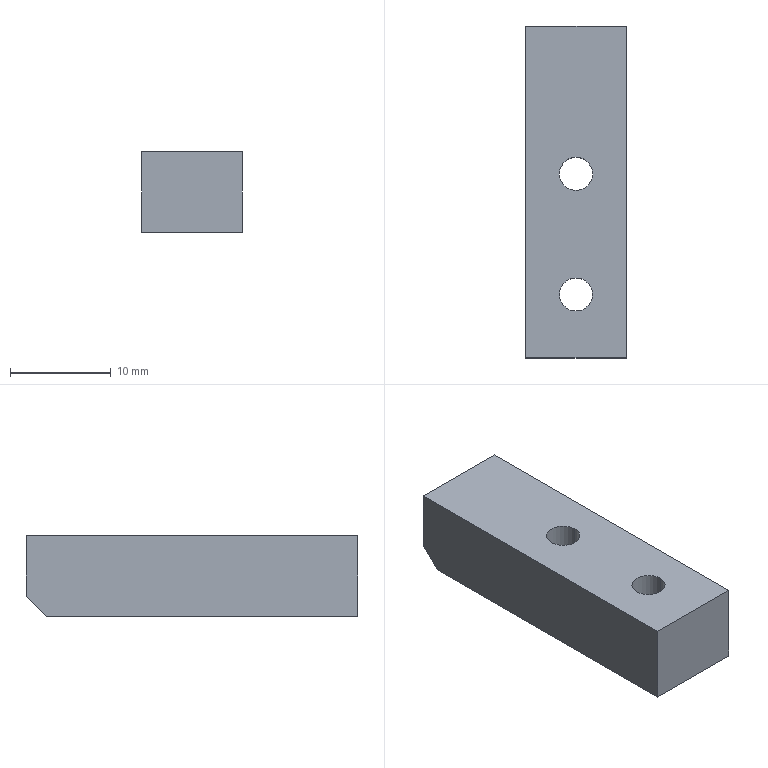Component | SolidWorks | 6G-TL06-StopBlock-2 | 1 solid | 11 faces | box 10 x 33 x 8 mm | volume 2483 mm3 | plane 7 | cylinder 4 | commonest cylinder face diameters 3.3 x4
build123d program:
from build123d import *

# Parameters (mm, degrees)
SKETCH1_W           = 33
SKETCH1_H           = 8
BOSS_EXTRUDE1_DEPTH = 10
M4_TAPPED_HOLE1_D   = 3.3
CHAMFER1_SIZE       = 2


with BuildPart() as part:
    # Sketch1 → Boss-Extrude1 (new body)
    with BuildSketch(Plane.XY):
        Rectangle(SKETCH1_W, SKETCH1_H)
    extrude(amount=-BOSS_EXTRUDE1_DEPTH)

    # M4 Tapped Hole1 (through all)
    with Locations(Plane(origin=(10.2, 4, -5), x_dir=(0, 0, 1), z_dir=(0, 1, 0))):
        with Locations((0, 0), (0, -12)):
            Hole(M4_TAPPED_HOLE1_D / 2)

    # Chamfer1
    chamfer1_edges = [part.edges().sort_by_distance(p)[0] for p in [
        (-16.5, -4, -5),
    ]]
    chamfer(chamfer1_edges, length=CHAMFER1_SIZE)


solid = part.part

# Placed as in the assembly
solid = solid.moved(Location((-113.5, 333.2, -29), (90, -90, 0)))
STEP:
#1=CARTESIAN_POINT('',(-4.207,12.717,-1.299));
#2=VERTEX_POINT('',#1);
#3=CARTESIAN_POINT('',(-4.337,12.717,-1.299));
#4=VERTEX_POINT('',#3);
#5=CARTESIAN_POINT('',(-4.272,12.717,-1.299));
#6=DIRECTION('',(-0.,-0.,1.));
#7=DIRECTION('',(-1.,0.,0.));
#8=AXIS2_PLACEMENT_3D('',#5,#6,#7);
#9=CIRCLE('',#8,0.06496);
#10=EDGE_CURVE('',#2,#4,#9,.T.);
#11=ORIENTED_EDGE('',*,*,#10,.F.);
#12=CARTESIAN_POINT('',(-4.207,12.717,-0.9843));
#13=VERTEX_POINT('',#12);
#14=CARTESIAN_POINT('',(-4.207,12.717,-0.9843));
#15=DIRECTION('',(-0.,-0.,1.));
#16=VECTOR('',#15,39.37);
#17=LINE('',#14,#16);
#18=EDGE_CURVE('',#2,#13,#17,.T.);
#19=ORIENTED_EDGE('',*,*,#18,.T.);
#20=CARTESIAN_POINT('',(-4.337,12.717,-0.9843));
#21=VERTEX_POINT('',#20);
#22=CARTESIAN_POINT('',(-4.272,12.717,-0.9843));
#23=DIRECTION('',(-0.,-0.,1.));
#24=DIRECTION('',(-1.,0.,0.));
#25=AXIS2_PLACEMENT_3D('',#22,#23,#24);
#26=CIRCLE('',#25,0.06496);
#27=EDGE_CURVE('',#13,#21,#26,.T.);
#28=ORIENTED_EDGE('',*,*,#27,.T.);
#29=CARTESIAN_POINT('',(-4.337,12.717,-0.9843));
#30=DIRECTION('',(-0.,-0.,1.));
#31=VECTOR('',#30,39.37);
#32=LINE('',#29,#31);
#33=EDGE_CURVE('',#4,#21,#32,.T.);
#34=ORIENTED_EDGE('',*,*,#33,.F.);
#35=EDGE_LOOP('',(#11,#19,#28,#34));
#36=FACE_OUTER_BOUND('',#35,.T.);
#37=CARTESIAN_POINT('',(-4.272,12.717,-0.9843));
#38=DIRECTION('',(-0.,-0.,1.));
#39=DIRECTION('',(-1.,0.,0.));
#40=AXIS2_PLACEMENT_3D('',#37,#38,#39);
#41=CYLINDRICAL_SURFACE('',#40,0.06496);
#42=ADVANCED_FACE('',(#36),#41,.F.);
#43=CARTESIAN_POINT('',(-4.207,13.189,-1.299));
#44=VERTEX_POINT('',#43);
#45=CARTESIAN_POINT('',(-4.337,13.189,-1.299));
#46=VERTEX_POINT('',#45);
#47=CARTESIAN_POINT('',(-4.272,13.189,-1.299));
#48=DIRECTION('',(-0.,-0.,1.));
#49=DIRECTION('',(-1.,0.,0.));
#50=AXIS2_PLACEMENT_3D('',#47,#48,#49);
#51=CIRCLE('',#50,0.06496);
#52=EDGE_CURVE('',#44,#46,#51,.T.);
#53=ORIENTED_EDGE('',*,*,#52,.F.);
#54=CARTESIAN_POINT('',(-4.207,13.189,-0.9843));
#55=VERTEX_POINT('',#54);
#56=CARTESIAN_POINT('',(-4.207,13.189,-0.9843));
#57=DIRECTION('',(-0.,-0.,1.));
#58=VECTOR('',#57,39.37);
#59=LINE('',#56,#58);
#60=EDGE_CURVE('',#44,#55,#59,.T.);
#61=ORIENTED_EDGE('',*,*,#60,.T.);
#62=CARTESIAN_POINT('',(-4.337,13.189,-0.9843));
#63=VERTEX_POINT('',#62);
#64=CARTESIAN_POINT('',(-4.272,13.189,-0.9843));
#65=DIRECTION('',(-0.,-0.,1.));
#66=DIRECTION('',(-1.,0.,0.));
#67=AXIS2_PLACEMENT_3D('',#64,#65,#66);
#68=CIRCLE('',#67,0.06496);
#69=EDGE_CURVE('',#55,#63,#68,.T.);
#70=ORIENTED_EDGE('',*,*,#69,.T.);
#71=CARTESIAN_POINT('',(-4.337,13.189,-0.9843));
#72=DIRECTION('',(-0.,-0.,1.));
#73=VECTOR('',#72,39.37);
#74=LINE('',#71,#73);
#75=EDGE_CURVE('',#46,#63,#74,.T.);
#76=ORIENTED_EDGE('',*,*,#75,.F.);
#77=EDGE_LOOP('',(#53,#61,#70,#76));
#78=FACE_OUTER_BOUND('',#77,.T.);
#79=CARTESIAN_POINT('',(-4.272,13.189,-0.9843));
#80=DIRECTION('',(-0.,-0.,1.));
#81=DIRECTION('',(-1.,0.,0.));
#82=AXIS2_PLACEMENT_3D('',#79,#80,#81);
#83=CYLINDRICAL_SURFACE('',#82,0.06496);
#84=ADVANCED_FACE('',(#78),#83,.F.);
#85=CARTESIAN_POINT('',(-4.469,12.469,-1.299));
#86=VERTEX_POINT('',#85);
#87=CARTESIAN_POINT('',(-4.469,12.469,-0.9843));
#88=VERTEX_POINT('',#87);
#89=CARTESIAN_POINT('',(-4.469,12.469,-1.299));
#90=DIRECTION('',(-0.,-0.,1.));
#91=VECTOR('',#90,39.37);
#92=LINE('',#89,#91);
#93=EDGE_CURVE('',#86,#88,#92,.T.);
#94=ORIENTED_EDGE('',*,*,#93,.F.);
#95=CARTESIAN_POINT('',(-4.075,12.469,-1.299));
#96=VERTEX_POINT('',#95);
#97=CARTESIAN_POINT('',(-4.075,12.469,-1.299));
#98=DIRECTION('',(-1.,-0.,-0.));
#99=VECTOR('',#98,39.37);
#100=LINE('',#97,#99);
#101=EDGE_CURVE('',#96,#86,#100,.T.);
#102=ORIENTED_EDGE('',*,*,#101,.F.);
#103=CARTESIAN_POINT('',(-4.075,12.469,-0.9843));
#104=VERTEX_POINT('',#103);
#105=CARTESIAN_POINT('',(-4.075,12.469,-1.299));
#106=DIRECTION('',(-0.,-0.,1.));
#107=VECTOR('',#106,39.37);
#108=LINE('',#105,#107);
#109=EDGE_CURVE('',#96,#104,#108,.T.);
#110=ORIENTED_EDGE('',*,*,#109,.T.);
#111=CARTESIAN_POINT('',(-4.075,12.469,-0.9843));
#112=DIRECTION('',(-1.,-0.,-0.));
#113=VECTOR('',#112,39.37);
#114=LINE('',#111,#113);
#115=EDGE_CURVE('',#104,#88,#114,.T.);
#116=ORIENTED_EDGE('',*,*,#115,.T.);
#117=EDGE_LOOP('',(#94,#102,#110,#116));
#118=FACE_OUTER_BOUND('',#117,.T.);
#119=CARTESIAN_POINT('',(-4.075,12.469,-1.299));
#120=DIRECTION('',(0.,-1.,-0.));
#121=DIRECTION('',(1.,0.,0.));
#122=AXIS2_PLACEMENT_3D('',#119,#120,#121);
#123=PLANE('',#122);
#124=ADVANCED_FACE('',(#118),#123,.T.);
#125=CARTESIAN_POINT('',(-4.272,12.717,-1.299));
#126=DIRECTION('',(-0.,-0.,1.));
#127=DIRECTION('',(-1.,0.,0.));
#128=AXIS2_PLACEMENT_3D('',#125,#126,#127);
#129=CIRCLE('',#128,0.06496);
#130=EDGE_CURVE('',#4,#2,#129,.T.);
#131=ORIENTED_EDGE('',*,*,#130,.T.);
#132=ORIENTED_EDGE('',*,*,#10,.T.);
#133=EDGE_LOOP('',(#131,#132));
#134=FACE_BOUND('',#133,.T.);
#135=CARTESIAN_POINT('',(-4.272,13.189,-1.299));
#136=DIRECTION('',(-0.,-0.,1.));
#137=DIRECTION('',(-1.,0.,0.));
#138=AXIS2_PLACEMENT_3D('',#135,#136,#137);
#139=CIRCLE('',#138,0.06496);
#140=EDGE_CURVE('',#46,#44,#139,.T.);
#141=ORIENTED_EDGE('',*,*,#140,.T.);
#142=ORIENTED_EDGE('',*,*,#52,.T.);
#143=EDGE_LOOP('',(#141,#142));
#144=FACE_BOUND('',#143,.T.);
#145=CARTESIAN_POINT('',(-4.469,13.689,-1.299));
#146=VERTEX_POINT('',#145);
#147=CARTESIAN_POINT('',(-4.469,13.768,-1.299));
#148=DIRECTION('',(0.,-1.,-0.));
#149=VECTOR('',#148,39.37);
#150=LINE('',#147,#149);
#151=EDGE_CURVE('',#146,#86,#150,.T.);
#152=ORIENTED_EDGE('',*,*,#151,.F.);
#153=CARTESIAN_POINT('',(-4.075,13.689,-1.299));
#154=VERTEX_POINT('',#153);
#155=CARTESIAN_POINT('',(-4.075,13.689,-1.299));
#156=DIRECTION('',(1.,0.,0.));
#157=VECTOR('',#156,39.37);
#158=LINE('',#155,#157);
#159=EDGE_CURVE('',#146,#154,#158,.T.);
#160=ORIENTED_EDGE('',*,*,#159,.T.);
#161=CARTESIAN_POINT('',(-4.075,13.768,-1.299));
#162=DIRECTION('',(0.,-1.,-0.));
#163=VECTOR('',#162,39.37);
#164=LINE('',#161,#163);
#165=EDGE_CURVE('',#154,#96,#164,.T.);
#166=ORIENTED_EDGE('',*,*,#165,.T.);
#167=ORIENTED_EDGE('',*,*,#101,.T.);
#168=EDGE_LOOP('',(#152,#160,#166,#167));
#169=FACE_OUTER_BOUND('',#168,.T.);
#170=CARTESIAN_POINT('',(-4.075,13.768,-1.299));
#171=DIRECTION('',(0.,0.,-1.));
#172=DIRECTION('',(1.,0.,0.));
#173=AXIS2_PLACEMENT_3D('',#170,#171,#172);
#174=PLANE('',#173);
#175=ADVANCED_FACE('',(#134,#144,#169),#174,.T.);
#176=CARTESIAN_POINT('',(-4.075,13.768,-0.9843));
#177=VERTEX_POINT('',#176);
#178=CARTESIAN_POINT('',(-4.075,13.768,-1.22));
#179=VERTEX_POINT('',#178);
#180=CARTESIAN_POINT('',(-4.075,13.768,-1.299));
#181=DIRECTION('',(0.,0.,-1.));
#182=VECTOR('',#181,39.37);
#183=LINE('',#180,#182);
#184=EDGE_CURVE('',#177,#179,#183,.T.);
#185=ORIENTED_EDGE('',*,*,#184,.T.);
#186=CARTESIAN_POINT('',(-4.469,13.768,-1.22));
#187=VERTEX_POINT('',#186);
#188=CARTESIAN_POINT('',(-4.075,13.768,-1.22));
#189=DIRECTION('',(-1.,-0.,-0.));
#190=VECTOR('',#189,39.37);
#191=LINE('',#188,#190);
#192=EDGE_CURVE('',#179,#187,#191,.T.);
#193=ORIENTED_EDGE('',*,*,#192,.T.);
#194=CARTESIAN_POINT('',(-4.469,13.768,-0.9843));
#195=VERTEX_POINT('',#194);
#196=CARTESIAN_POINT('',(-4.469,13.768,-1.299));
#197=DIRECTION('',(0.,0.,-1.));
#198=VECTOR('',#197,39.37);
#199=LINE('',#196,#198);
#200=EDGE_CURVE('',#195,#187,#199,.T.);
#201=ORIENTED_EDGE('',*,*,#200,.F.);
#202=CARTESIAN_POINT('',(-4.075,13.768,-0.9843));
#203=DIRECTION('',(-1.,-0.,-0.));
#204=VECTOR('',#203,39.37);
#205=LINE('',#202,#204);
#206=EDGE_CURVE('',#177,#195,#205,.T.);
#207=ORIENTED_EDGE('',*,*,#206,.F.);
#208=EDGE_LOOP('',(#185,#193,#201,#207));
#209=FACE_OUTER_BOUND('',#208,.T.);
#210=CARTESIAN_POINT('',(-4.075,13.768,-1.299));
#211=DIRECTION('',(-0.,1.,0.));
#212=DIRECTION('',(-1.,-0.,-0.));
#213=AXIS2_PLACEMENT_3D('',#210,#211,#212);
#214=PLANE('',#213);
#215=ADVANCED_FACE('',(#209),#214,.T.);
#216=CARTESIAN_POINT('',(-4.272,12.717,-0.9843));
#217=DIRECTION('',(-0.,-0.,1.));
#218=DIRECTION('',(-1.,0.,0.));
#219=AXIS2_PLACEMENT_3D('',#216,#217,#218);
#220=CIRCLE('',#219,0.06496);
#221=EDGE_CURVE('',#21,#13,#220,.T.);
#222=ORIENTED_EDGE('',*,*,#221,.F.);
#223=ORIENTED_EDGE('',*,*,#27,.F.);
#224=EDGE_LOOP('',(#222,#223));
#225=FACE_BOUND('',#224,.T.);
#226=CARTESIAN_POINT('',(-4.272,13.189,-0.9843));
#227=DIRECTION('',(-0.,-0.,1.));
#228=DIRECTION('',(-1.,0.,0.));
#229=AXIS2_PLACEMENT_3D('',#226,#227,#228);
#230=CIRCLE('',#229,0.06496);
#231=EDGE_CURVE('',#63,#55,#230,.T.);
#232=ORIENTED_EDGE('',*,*,#231,.F.);
#233=ORIENTED_EDGE('',*,*,#69,.F.);
#234=EDGE_LOOP('',(#232,#233));
#235=FACE_BOUND('',#234,.T.);
#236=CARTESIAN_POINT('',(-4.469,13.768,-0.9843));
#237=DIRECTION('',(-0.,1.,0.));
#238=VECTOR('',#237,39.37);
#239=LINE('',#236,#238);
#240=EDGE_CURVE('',#88,#195,#239,.T.);
#241=ORIENTED_EDGE('',*,*,#240,.F.);
#242=ORIENTED_EDGE('',*,*,#115,.F.);
#243=CARTESIAN_POINT('',(-4.075,13.768,-0.9843));
#244=DIRECTION('',(-0.,1.,0.));
#245=VECTOR('',#244,39.37);
#246=LINE('',#243,#245);
#247=EDGE_CURVE('',#104,#177,#246,.T.);
#248=ORIENTED_EDGE('',*,*,#247,.T.);
#249=ORIENTED_EDGE('',*,*,#206,.T.);
#250=EDGE_LOOP('',(#241,#242,#248,#249));
#251=FACE_OUTER_BOUND('',#250,.T.);
#252=CARTESIAN_POINT('',(-4.075,13.768,-0.9843));
#253=DIRECTION('',(-0.,-0.,1.));
#254=DIRECTION('',(-1.,-0.,-0.));
#255=AXIS2_PLACEMENT_3D('',#252,#253,#254);
#256=PLANE('',#255);
#257=ADVANCED_FACE('',(#225,#235,#251),#256,.T.);
#258=ORIENTED_EDGE('',*,*,#165,.F.);
#259=CARTESIAN_POINT('',(-4.075,13.482,-1.506));
#260=DIRECTION('',(-0.,0.7071,0.7071));
#261=VECTOR('',#260,39.37);
#262=LINE('',#259,#261);
#263=EDGE_CURVE('',#154,#179,#262,.T.);
#264=ORIENTED_EDGE('',*,*,#263,.T.);
#265=ORIENTED_EDGE('',*,*,#184,.F.);
#266=ORIENTED_EDGE('',*,*,#247,.F.);
#267=ORIENTED_EDGE('',*,*,#109,.F.);
#268=EDGE_LOOP('',(#258,#264,#265,#266,#267));
#269=FACE_OUTER_BOUND('',#268,.T.);
#270=CARTESIAN_POINT('',(-4.075,13.118,-1.142));
#271=DIRECTION('',(1.,0.,0.));
#272=DIRECTION('',(-0.,1.,0.));
#273=AXIS2_PLACEMENT_3D('',#270,#271,#272);
#274=PLANE('',#273);
#275=ADVANCED_FACE('',(#269),#274,.T.);
#276=ORIENTED_EDGE('',*,*,#200,.T.);
#277=CARTESIAN_POINT('',(-4.469,13.768,-1.22));
#278=DIRECTION('',(0.,-0.7071,-0.7071));
#279=VECTOR('',#278,39.37);
#280=LINE('',#277,#279);
#281=EDGE_CURVE('',#187,#146,#280,.T.);
#282=ORIENTED_EDGE('',*,*,#281,.T.);
#283=ORIENTED_EDGE('',*,*,#151,.T.);
#284=ORIENTED_EDGE('',*,*,#93,.T.);
#285=ORIENTED_EDGE('',*,*,#240,.T.);
#286=EDGE_LOOP('',(#276,#282,#283,#284,#285));
#287=FACE_OUTER_BOUND('',#286,.T.);
#288=CARTESIAN_POINT('',(-4.469,13.118,-1.142));
#289=DIRECTION('',(1.,0.,0.));
#290=DIRECTION('',(-0.,1.,0.));
#291=AXIS2_PLACEMENT_3D('',#288,#289,#290);
#292=PLANE('',#291);
#293=ADVANCED_FACE('',(#287),#292,.F.);
#294=ORIENTED_EDGE('',*,*,#60,.F.);
#295=ORIENTED_EDGE('',*,*,#140,.F.);
#296=ORIENTED_EDGE('',*,*,#75,.T.);
#297=ORIENTED_EDGE('',*,*,#231,.T.);
#298=EDGE_LOOP('',(#294,#295,#296,#297));
#299=FACE_OUTER_BOUND('',#298,.T.);
#300=CARTESIAN_POINT('',(-4.272,13.189,-0.9843));
#301=DIRECTION('',(-0.,-0.,1.));
#302=DIRECTION('',(-1.,0.,0.));
#303=AXIS2_PLACEMENT_3D('',#300,#301,#302);
#304=CYLINDRICAL_SURFACE('',#303,0.06496);
#305=ADVANCED_FACE('',(#299),#304,.F.);
#306=ORIENTED_EDGE('',*,*,#18,.F.);
#307=ORIENTED_EDGE('',*,*,#130,.F.);
#308=ORIENTED_EDGE('',*,*,#33,.T.);
#309=ORIENTED_EDGE('',*,*,#221,.T.);
#310=EDGE_LOOP('',(#306,#307,#308,#309));
#311=FACE_OUTER_BOUND('',#310,.T.);
#312=CARTESIAN_POINT('',(-4.272,12.717,-0.9843));
#313=DIRECTION('',(-0.,-0.,1.));
#314=DIRECTION('',(-1.,0.,0.));
#315=AXIS2_PLACEMENT_3D('',#312,#313,#314);
#316=CYLINDRICAL_SURFACE('',#315,0.06496);
#317=ADVANCED_FACE('',(#311),#316,.F.);
#318=ORIENTED_EDGE('',*,*,#263,.F.);
#319=ORIENTED_EDGE('',*,*,#159,.F.);
#320=ORIENTED_EDGE('',*,*,#281,.F.);
#321=ORIENTED_EDGE('',*,*,#192,.F.);
#322=EDGE_LOOP('',(#318,#319,#320,#321));
#323=FACE_OUTER_BOUND('',#322,.T.);
#324=CARTESIAN_POINT('',(-4.075,13.768,-1.22));
#325=DIRECTION('',(0.,-0.7071,0.7071));
#326=DIRECTION('',(-1.,-0.,-0.));
#327=AXIS2_PLACEMENT_3D('',#324,#325,#326);
#328=PLANE('',#327);
#329=ADVANCED_FACE('',(#323),#328,.F.);
#330=CLOSED_SHELL('',(#42,#84,#124,#175,#215,#257,#275,#293,#305,#317,#329));
#331=MANIFOLD_SOLID_BREP('',#330);
#332=CARTESIAN_POINT('',(0.,0.,0.));
#333=DIRECTION('',(0.,0.,1.));
#334=DIRECTION('',(1.,0.,0.));
#335=AXIS2_PLACEMENT_3D('',#332,#333,#334);
#336=(LENGTH_UNIT()NAMED_UNIT(*)SI_UNIT($,.METRE.));
#337=LENGTH_MEASURE_WITH_UNIT(LENGTH_MEASURE(0.0254),#336);
#338=DIMENSIONAL_EXPONENTS(1.,0.,0.,0.,0.,0.,0.);
#339=(CONVERSION_BASED_UNIT('',#337)LENGTH_UNIT()NAMED_UNIT(#338));
#340=UNCERTAINTY_MEASURE_WITH_UNIT(LENGTH_MEASURE(0.00001),#339,'','');
#341=(NAMED_UNIT(*)PLANE_ANGLE_UNIT()SI_UNIT($,.RADIAN.));
#342=(NAMED_UNIT(*)SI_UNIT($,.STERADIAN.)SOLID_ANGLE_UNIT());
#343=(GEOMETRIC_REPRESENTATION_CONTEXT(3)GLOBAL_UNCERTAINTY_ASSIGNED_CONTEXT((#340))GLOBAL_UNIT_ASSIGNED_CONTEXT((#339,#341,#342))REPRESENTATION_CONTEXT('',''));
#344=ADVANCED_BREP_SHAPE_REPRESENTATION('',(#331,#335),#343);
#345=COLOUR_RGB('',0.7922,0.8196,0.9333);
#346=FILL_AREA_STYLE_COLOUR('',#345);
#347=FILL_AREA_STYLE('',(#346));
#348=SURFACE_STYLE_FILL_AREA(#347);
#349=SURFACE_SIDE_STYLE('',(#348));
#350=SURFACE_STYLE_USAGE(.BOTH.,#349);
#351=PRESENTATION_STYLE_ASSIGNMENT((#350));
#352=STYLED_ITEM('',(#351),#331);
#353=(LENGTH_UNIT()NAMED_UNIT(*)SI_UNIT($,.METRE.));
#354=LENGTH_MEASURE_WITH_UNIT(LENGTH_MEASURE(0.0254),#353);
#355=DIMENSIONAL_EXPONENTS(1.,0.,0.,0.,0.,0.,0.);
#356=(CONVERSION_BASED_UNIT('',#354)LENGTH_UNIT()NAMED_UNIT(#355));
#357=UNCERTAINTY_MEASURE_WITH_UNIT(LENGTH_MEASURE(0.00001),#356,'','');
#358=(NAMED_UNIT(*)PLANE_ANGLE_UNIT()SI_UNIT($,.RADIAN.));
#359=(NAMED_UNIT(*)SI_UNIT($,.STERADIAN.)SOLID_ANGLE_UNIT());
#360=(GEOMETRIC_REPRESENTATION_CONTEXT(3)GLOBAL_UNCERTAINTY_ASSIGNED_CONTEXT((#357))GLOBAL_UNIT_ASSIGNED_CONTEXT((#356,#358,#359))REPRESENTATION_CONTEXT('',''));
#361=MECHANICAL_DESIGN_GEOMETRIC_PRESENTATION_REPRESENTATION('',(#352),#360);
#362=PRESENTATION_LAYER_ASSIGNMENT('','',(#352));